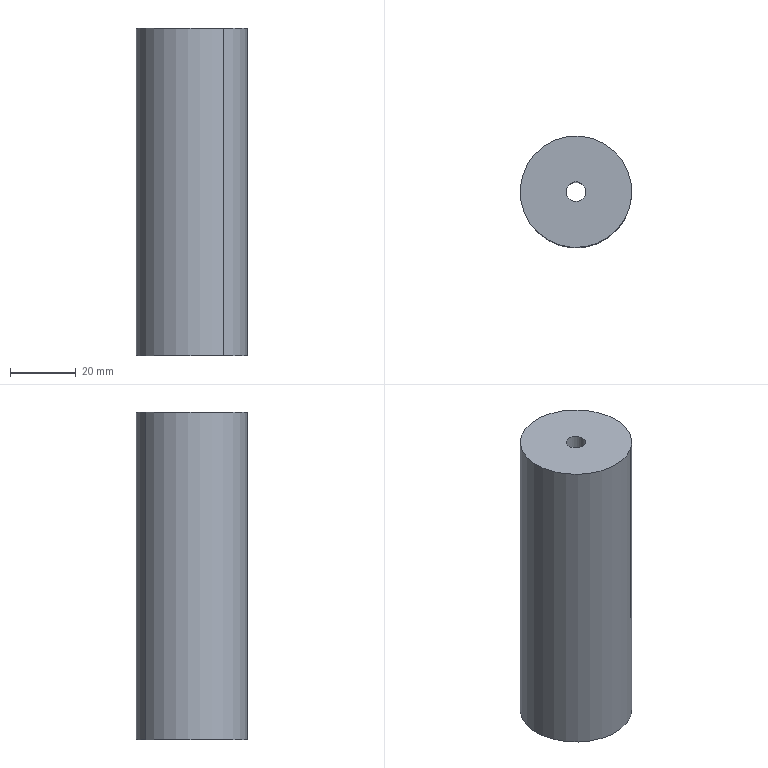Component | SolidWorks | TrackDriveStrip-2 | 1 solid | 6 faces | box 34 x 34 x 100 mm | volume 87965 mm3 | cylinder 4 | plane 2 | commonest cylinder face diameters 6 x2 34 x2
build123d program:
from build123d import *

# Parameters (mm, degrees)
SKETCH1_R           = 17
SKETCH1_R_2         = 3
BOSS_EXTRUDE1_DEPTH = 100


with BuildPart() as part:
    # Sketch1 → Boss-Extrude1 (new body)
    with BuildSketch(Plane.XY):
        with Locations((71.434, 305)):
            Circle(SKETCH1_R)
        with Locations((71.434, 305)):
            Circle(SKETCH1_R_2, mode=Mode.SUBTRACT)
    extrude(amount=-BOSS_EXTRUDE1_DEPTH)


solid = part.part

# Placed as in the assembly
solid = solid.moved(Location((-511.434, -213, 50), (0, 0, 0)))
STEP:
#1=COLOUR_RGB('',0.7922,0.8196,0.9333);
#2=FILL_AREA_STYLE_COLOUR('',#1);
#3=FILL_AREA_STYLE('',(#2));
#4=SURFACE_STYLE_FILL_AREA(#3);
#5=SURFACE_SIDE_STYLE('',(#4));
#6=SURFACE_STYLE_USAGE(.BOTH.,#5);
#7=PRESENTATION_STYLE_ASSIGNMENT((#6));
#8=CARTESIAN_POINT('',(-17.256,3.525,-1.969));
#9=VERTEX_POINT('',#8);
#10=CARTESIAN_POINT('',(-17.389,3.72,-1.969));
#11=VERTEX_POINT('',#10);
#12=CARTESIAN_POINT('',(-17.323,3.622,-1.969));
#13=DIRECTION('',(0.,0.,1.));
#14=DIRECTION('',(-0.5642,0.8257,0.));
#15=AXIS2_PLACEMENT_3D('',#12,#13,#14);
#16=CIRCLE('',#15,0.1181);
#17=EDGE_CURVE('',#9,#11,#16,.T.);
#18=ORIENTED_EDGE('',*,*,#17,.F.);
#19=CARTESIAN_POINT('',(-17.256,3.525,1.969));
#20=VERTEX_POINT('',#19);
#21=CARTESIAN_POINT('',(-17.256,3.525,-1.969));
#22=DIRECTION('',(0.,0.,1.));
#23=VECTOR('',#22,39.37);
#24=LINE('',#21,#23);
#25=EDGE_CURVE('',#9,#20,#24,.T.);
#26=ORIENTED_EDGE('',*,*,#25,.T.);
#27=CARTESIAN_POINT('',(-17.389,3.72,1.969));
#28=VERTEX_POINT('',#27);
#29=CARTESIAN_POINT('',(-17.323,3.622,1.969));
#30=DIRECTION('',(0.,0.,1.));
#31=DIRECTION('',(-0.5642,0.8257,0.));
#32=AXIS2_PLACEMENT_3D('',#29,#30,#31);
#33=CIRCLE('',#32,0.1181);
#34=EDGE_CURVE('',#20,#28,#33,.T.);
#35=ORIENTED_EDGE('',*,*,#34,.T.);
#36=CARTESIAN_POINT('',(-17.389,3.72,-1.969));
#37=DIRECTION('',(0.,0.,1.));
#38=VECTOR('',#37,39.37);
#39=LINE('',#36,#38);
#40=EDGE_CURVE('',#11,#28,#39,.T.);
#41=ORIENTED_EDGE('',*,*,#40,.F.);
#42=EDGE_LOOP('',(#18,#26,#35,#41));
#43=FACE_OUTER_BOUND('',#42,.T.);
#44=CARTESIAN_POINT('',(-17.323,3.622,-1.969));
#45=DIRECTION('',(0.,0.,1.));
#46=DIRECTION('',(-0.5642,0.8257,0.));
#47=AXIS2_PLACEMENT_3D('',#44,#45,#46);
#48=CYLINDRICAL_SURFACE('',#47,0.1181);
#49=ADVANCED_FACE('',(#43),#48,.F.);
#50=CARTESIAN_POINT('',(-17.7,4.175,-1.969));
#51=VERTEX_POINT('',#50);
#52=CARTESIAN_POINT('',(-16.945,3.069,-1.969));
#53=VERTEX_POINT('',#52);
#54=CARTESIAN_POINT('',(-17.323,3.622,-1.969));
#55=DIRECTION('',(0.,0.,1.));
#56=DIRECTION('',(-0.5642,0.8257,0.));
#57=AXIS2_PLACEMENT_3D('',#54,#55,#56);
#58=CIRCLE('',#57,0.6693);
#59=EDGE_CURVE('',#51,#53,#58,.T.);
#60=ORIENTED_EDGE('',*,*,#59,.T.);
#61=CARTESIAN_POINT('',(-16.945,3.069,1.969));
#62=VERTEX_POINT('',#61);
#63=CARTESIAN_POINT('',(-16.945,3.069,-1.969));
#64=DIRECTION('',(0.,0.,1.));
#65=VECTOR('',#64,39.37);
#66=LINE('',#63,#65);
#67=EDGE_CURVE('',#53,#62,#66,.T.);
#68=ORIENTED_EDGE('',*,*,#67,.T.);
#69=CARTESIAN_POINT('',(-17.7,4.175,1.969));
#70=VERTEX_POINT('',#69);
#71=CARTESIAN_POINT('',(-17.323,3.622,1.969));
#72=DIRECTION('',(0.,0.,1.));
#73=DIRECTION('',(-0.5642,0.8257,0.));
#74=AXIS2_PLACEMENT_3D('',#71,#72,#73);
#75=CIRCLE('',#74,0.6693);
#76=EDGE_CURVE('',#70,#62,#75,.T.);
#77=ORIENTED_EDGE('',*,*,#76,.F.);
#78=CARTESIAN_POINT('',(-17.7,4.175,-1.969));
#79=DIRECTION('',(0.,0.,1.));
#80=VECTOR('',#79,39.37);
#81=LINE('',#78,#80);
#82=EDGE_CURVE('',#51,#70,#81,.T.);
#83=ORIENTED_EDGE('',*,*,#82,.F.);
#84=EDGE_LOOP('',(#60,#68,#77,#83));
#85=FACE_OUTER_BOUND('',#84,.T.);
#86=CARTESIAN_POINT('',(-17.323,3.622,-1.969));
#87=DIRECTION('',(0.,0.,1.));
#88=DIRECTION('',(-0.5642,0.8257,0.));
#89=AXIS2_PLACEMENT_3D('',#86,#87,#88);
#90=CYLINDRICAL_SURFACE('',#89,0.6693);
#91=ADVANCED_FACE('',(#85),#90,.T.);
#92=ORIENTED_EDGE('',*,*,#67,.F.);
#93=CARTESIAN_POINT('',(-17.323,3.622,-1.969));
#94=DIRECTION('',(0.,0.,1.));
#95=DIRECTION('',(-0.5642,0.8257,0.));
#96=AXIS2_PLACEMENT_3D('',#93,#94,#95);
#97=CIRCLE('',#96,0.6693);
#98=EDGE_CURVE('',#53,#51,#97,.T.);
#99=ORIENTED_EDGE('',*,*,#98,.T.);
#100=ORIENTED_EDGE('',*,*,#82,.T.);
#101=CARTESIAN_POINT('',(-17.323,3.622,1.969));
#102=DIRECTION('',(0.,0.,1.));
#103=DIRECTION('',(-0.5642,0.8257,0.));
#104=AXIS2_PLACEMENT_3D('',#101,#102,#103);
#105=CIRCLE('',#104,0.6693);
#106=EDGE_CURVE('',#62,#70,#105,.T.);
#107=ORIENTED_EDGE('',*,*,#106,.F.);
#108=EDGE_LOOP('',(#92,#99,#100,#107));
#109=FACE_OUTER_BOUND('',#108,.T.);
#110=CARTESIAN_POINT('',(-17.323,3.622,-1.969));
#111=DIRECTION('',(0.,0.,1.));
#112=DIRECTION('',(-0.5642,0.8257,0.));
#113=AXIS2_PLACEMENT_3D('',#110,#111,#112);
#114=CYLINDRICAL_SURFACE('',#113,0.6693);
#115=ADVANCED_FACE('',(#109),#114,.T.);
#116=CARTESIAN_POINT('',(-17.323,3.622,-1.969));
#117=DIRECTION('',(0.,0.,1.));
#118=DIRECTION('',(-0.5642,0.8257,0.));
#119=AXIS2_PLACEMENT_3D('',#116,#117,#118);
#120=CIRCLE('',#119,0.1181);
#121=EDGE_CURVE('',#11,#9,#120,.T.);
#122=ORIENTED_EDGE('',*,*,#121,.T.);
#123=ORIENTED_EDGE('',*,*,#17,.T.);
#124=EDGE_LOOP('',(#122,#123));
#125=FACE_BOUND('',#124,.T.);
#126=ORIENTED_EDGE('',*,*,#59,.F.);
#127=ORIENTED_EDGE('',*,*,#98,.F.);
#128=EDGE_LOOP('',(#126,#127));
#129=FACE_OUTER_BOUND('',#128,.T.);
#130=CARTESIAN_POINT('',(-17.323,3.622,-1.969));
#131=DIRECTION('',(0.,0.,1.));
#132=DIRECTION('',(-0.5642,0.8257,0.));
#133=AXIS2_PLACEMENT_3D('',#130,#131,#132);
#134=PLANE('',#133);
#135=ADVANCED_FACE('',(#125,#129),#134,.F.);
#136=CARTESIAN_POINT('',(-17.323,3.622,1.969));
#137=DIRECTION('',(0.,0.,1.));
#138=DIRECTION('',(-0.5642,0.8257,0.));
#139=AXIS2_PLACEMENT_3D('',#136,#137,#138);
#140=CIRCLE('',#139,0.1181);
#141=EDGE_CURVE('',#28,#20,#140,.T.);
#142=ORIENTED_EDGE('',*,*,#141,.F.);
#143=ORIENTED_EDGE('',*,*,#34,.F.);
#144=EDGE_LOOP('',(#142,#143));
#145=FACE_BOUND('',#144,.T.);
#146=ORIENTED_EDGE('',*,*,#76,.T.);
#147=ORIENTED_EDGE('',*,*,#106,.T.);
#148=EDGE_LOOP('',(#146,#147));
#149=FACE_OUTER_BOUND('',#148,.T.);
#150=CARTESIAN_POINT('',(-17.323,3.622,1.969));
#151=DIRECTION('',(0.,0.,1.));
#152=DIRECTION('',(-0.5642,0.8257,0.));
#153=AXIS2_PLACEMENT_3D('',#150,#151,#152);
#154=PLANE('',#153);
#155=ADVANCED_FACE('',(#145,#149),#154,.T.);
#156=ORIENTED_EDGE('',*,*,#25,.F.);
#157=ORIENTED_EDGE('',*,*,#121,.F.);
#158=ORIENTED_EDGE('',*,*,#40,.T.);
#159=ORIENTED_EDGE('',*,*,#141,.T.);
#160=EDGE_LOOP('',(#156,#157,#158,#159));
#161=FACE_OUTER_BOUND('',#160,.T.);
#162=CARTESIAN_POINT('',(-17.323,3.622,-1.969));
#163=DIRECTION('',(0.,0.,1.));
#164=DIRECTION('',(-0.5642,0.8257,0.));
#165=AXIS2_PLACEMENT_3D('',#162,#163,#164);
#166=CYLINDRICAL_SURFACE('',#165,0.1181);
#167=ADVANCED_FACE('',(#161),#166,.F.);
#168=CLOSED_SHELL('',(#49,#91,#115,#135,#155,#167));
#169=MANIFOLD_SOLID_BREP('',#168);
#170=STYLED_ITEM('',(#7),#169);
#171=(LENGTH_UNIT()NAMED_UNIT(*)SI_UNIT($,.METRE.));
#172=LENGTH_MEASURE_WITH_UNIT(LENGTH_MEASURE(0.0254),#171);
#173=DIMENSIONAL_EXPONENTS(1.,0.,0.,0.,0.,0.,0.);
#174=(CONVERSION_BASED_UNIT('',#172)LENGTH_UNIT()NAMED_UNIT(#173));
#175=UNCERTAINTY_MEASURE_WITH_UNIT(LENGTH_MEASURE(0.00001),#174,'','');
#176=(NAMED_UNIT(*)PLANE_ANGLE_UNIT()SI_UNIT($,.RADIAN.));
#177=(NAMED_UNIT(*)SI_UNIT($,.STERADIAN.)SOLID_ANGLE_UNIT());
#178=(GEOMETRIC_REPRESENTATION_CONTEXT(3)GLOBAL_UNCERTAINTY_ASSIGNED_CONTEXT((#175))GLOBAL_UNIT_ASSIGNED_CONTEXT((#174,#176,#177))REPRESENTATION_CONTEXT('',''));
#179=MECHANICAL_DESIGN_GEOMETRIC_PRESENTATION_REPRESENTATION('',(#170),#178);
#180=PRESENTATION_LAYER_ASSIGNMENT('','',(#170));
#181=CARTESIAN_POINT('',(0.,0.,0.));
#182=DIRECTION('',(0.,0.,1.));
#183=DIRECTION('',(1.,0.,0.));
#184=AXIS2_PLACEMENT_3D('',#181,#182,#183);
#185=(LENGTH_UNIT()NAMED_UNIT(*)SI_UNIT($,.METRE.));
#186=LENGTH_MEASURE_WITH_UNIT(LENGTH_MEASURE(0.0254),#185);
#187=DIMENSIONAL_EXPONENTS(1.,0.,0.,0.,0.,0.,0.);
#188=(CONVERSION_BASED_UNIT('',#186)LENGTH_UNIT()NAMED_UNIT(#187));
#189=UNCERTAINTY_MEASURE_WITH_UNIT(LENGTH_MEASURE(0.00001),#188,'','');
#190=(NAMED_UNIT(*)PLANE_ANGLE_UNIT()SI_UNIT($,.RADIAN.));
#191=(NAMED_UNIT(*)SI_UNIT($,.STERADIAN.)SOLID_ANGLE_UNIT());
#192=(GEOMETRIC_REPRESENTATION_CONTEXT(3)GLOBAL_UNCERTAINTY_ASSIGNED_CONTEXT((#189))GLOBAL_UNIT_ASSIGNED_CONTEXT((#188,#190,#191))REPRESENTATION_CONTEXT('',''));
#193=ADVANCED_BREP_SHAPE_REPRESENTATION('',(#169,#184),#192);